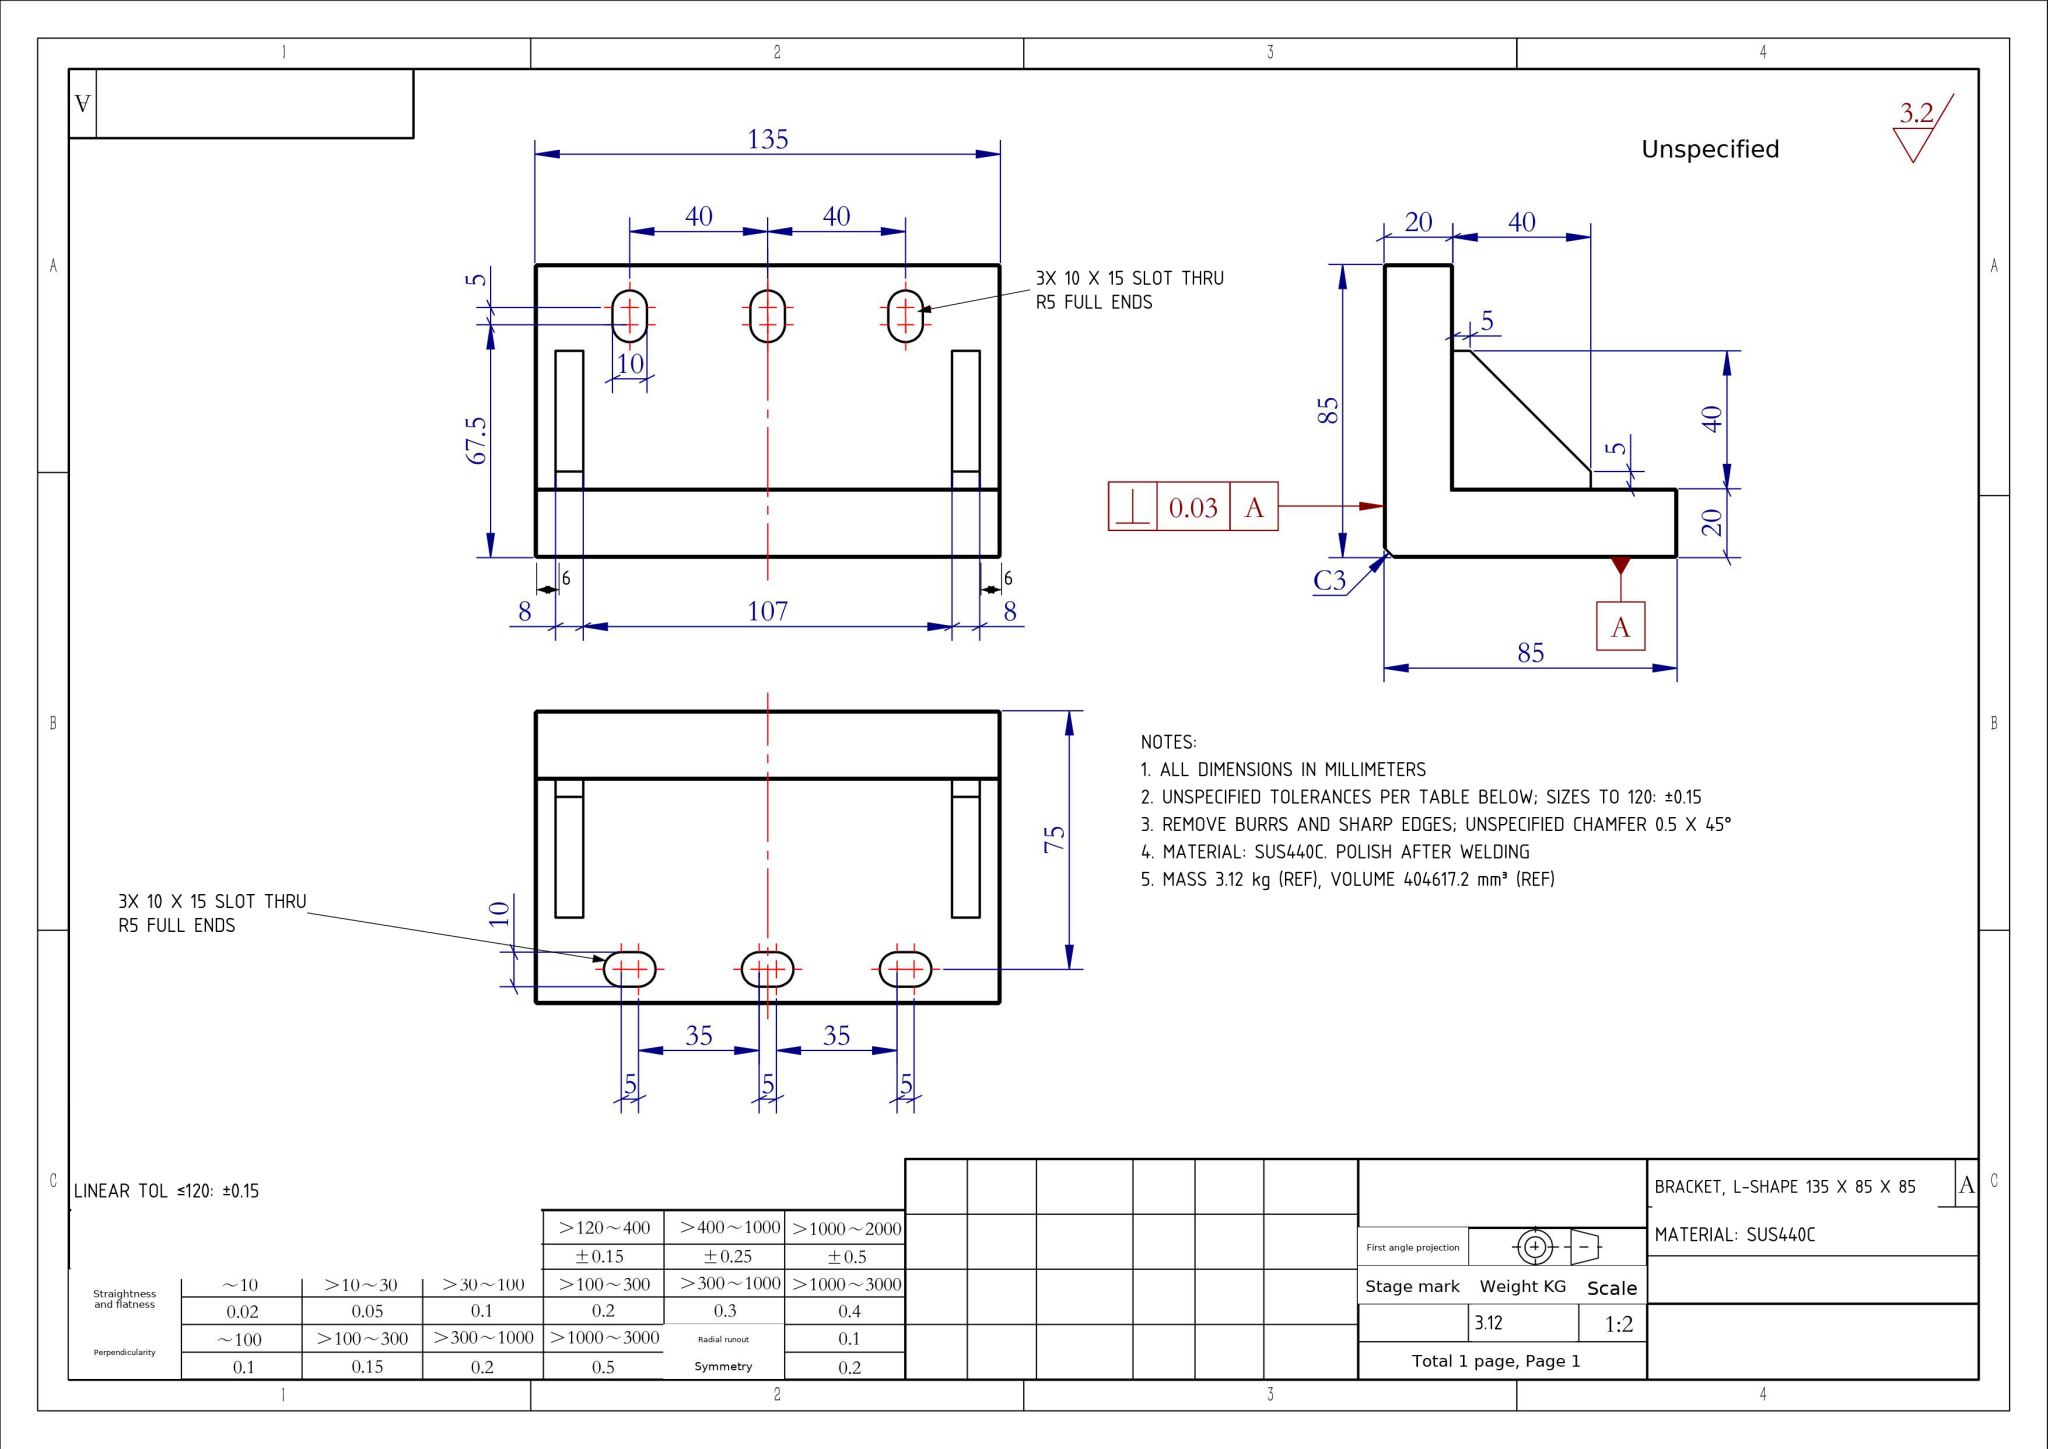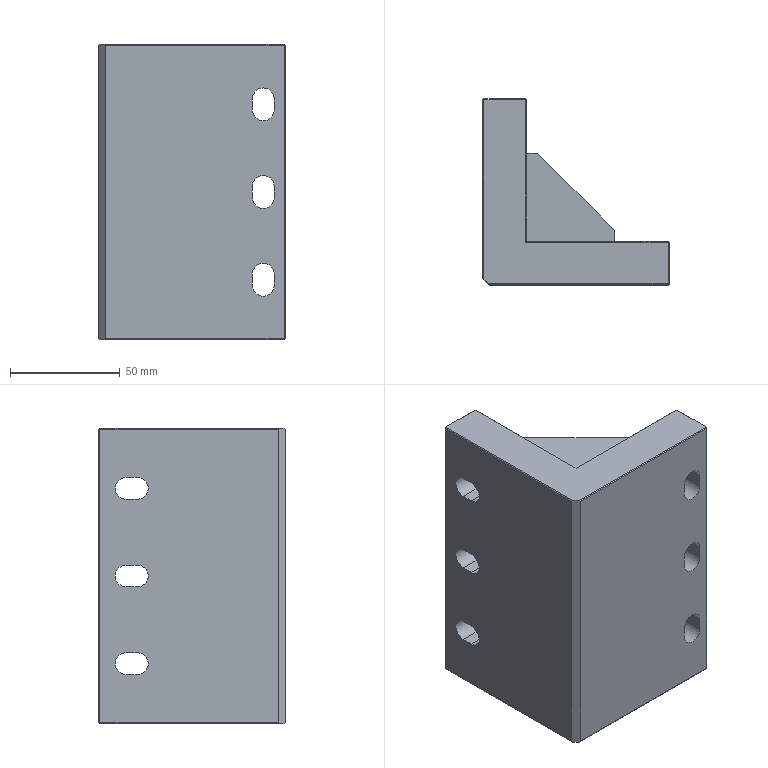Part | NX | mm | 1 solid | 70 faces | box 85 x 85 x 135 mm | volume 404617 mm3 | plane 55 | cylinder 15 | commonest cylinder face diameters 10 x15